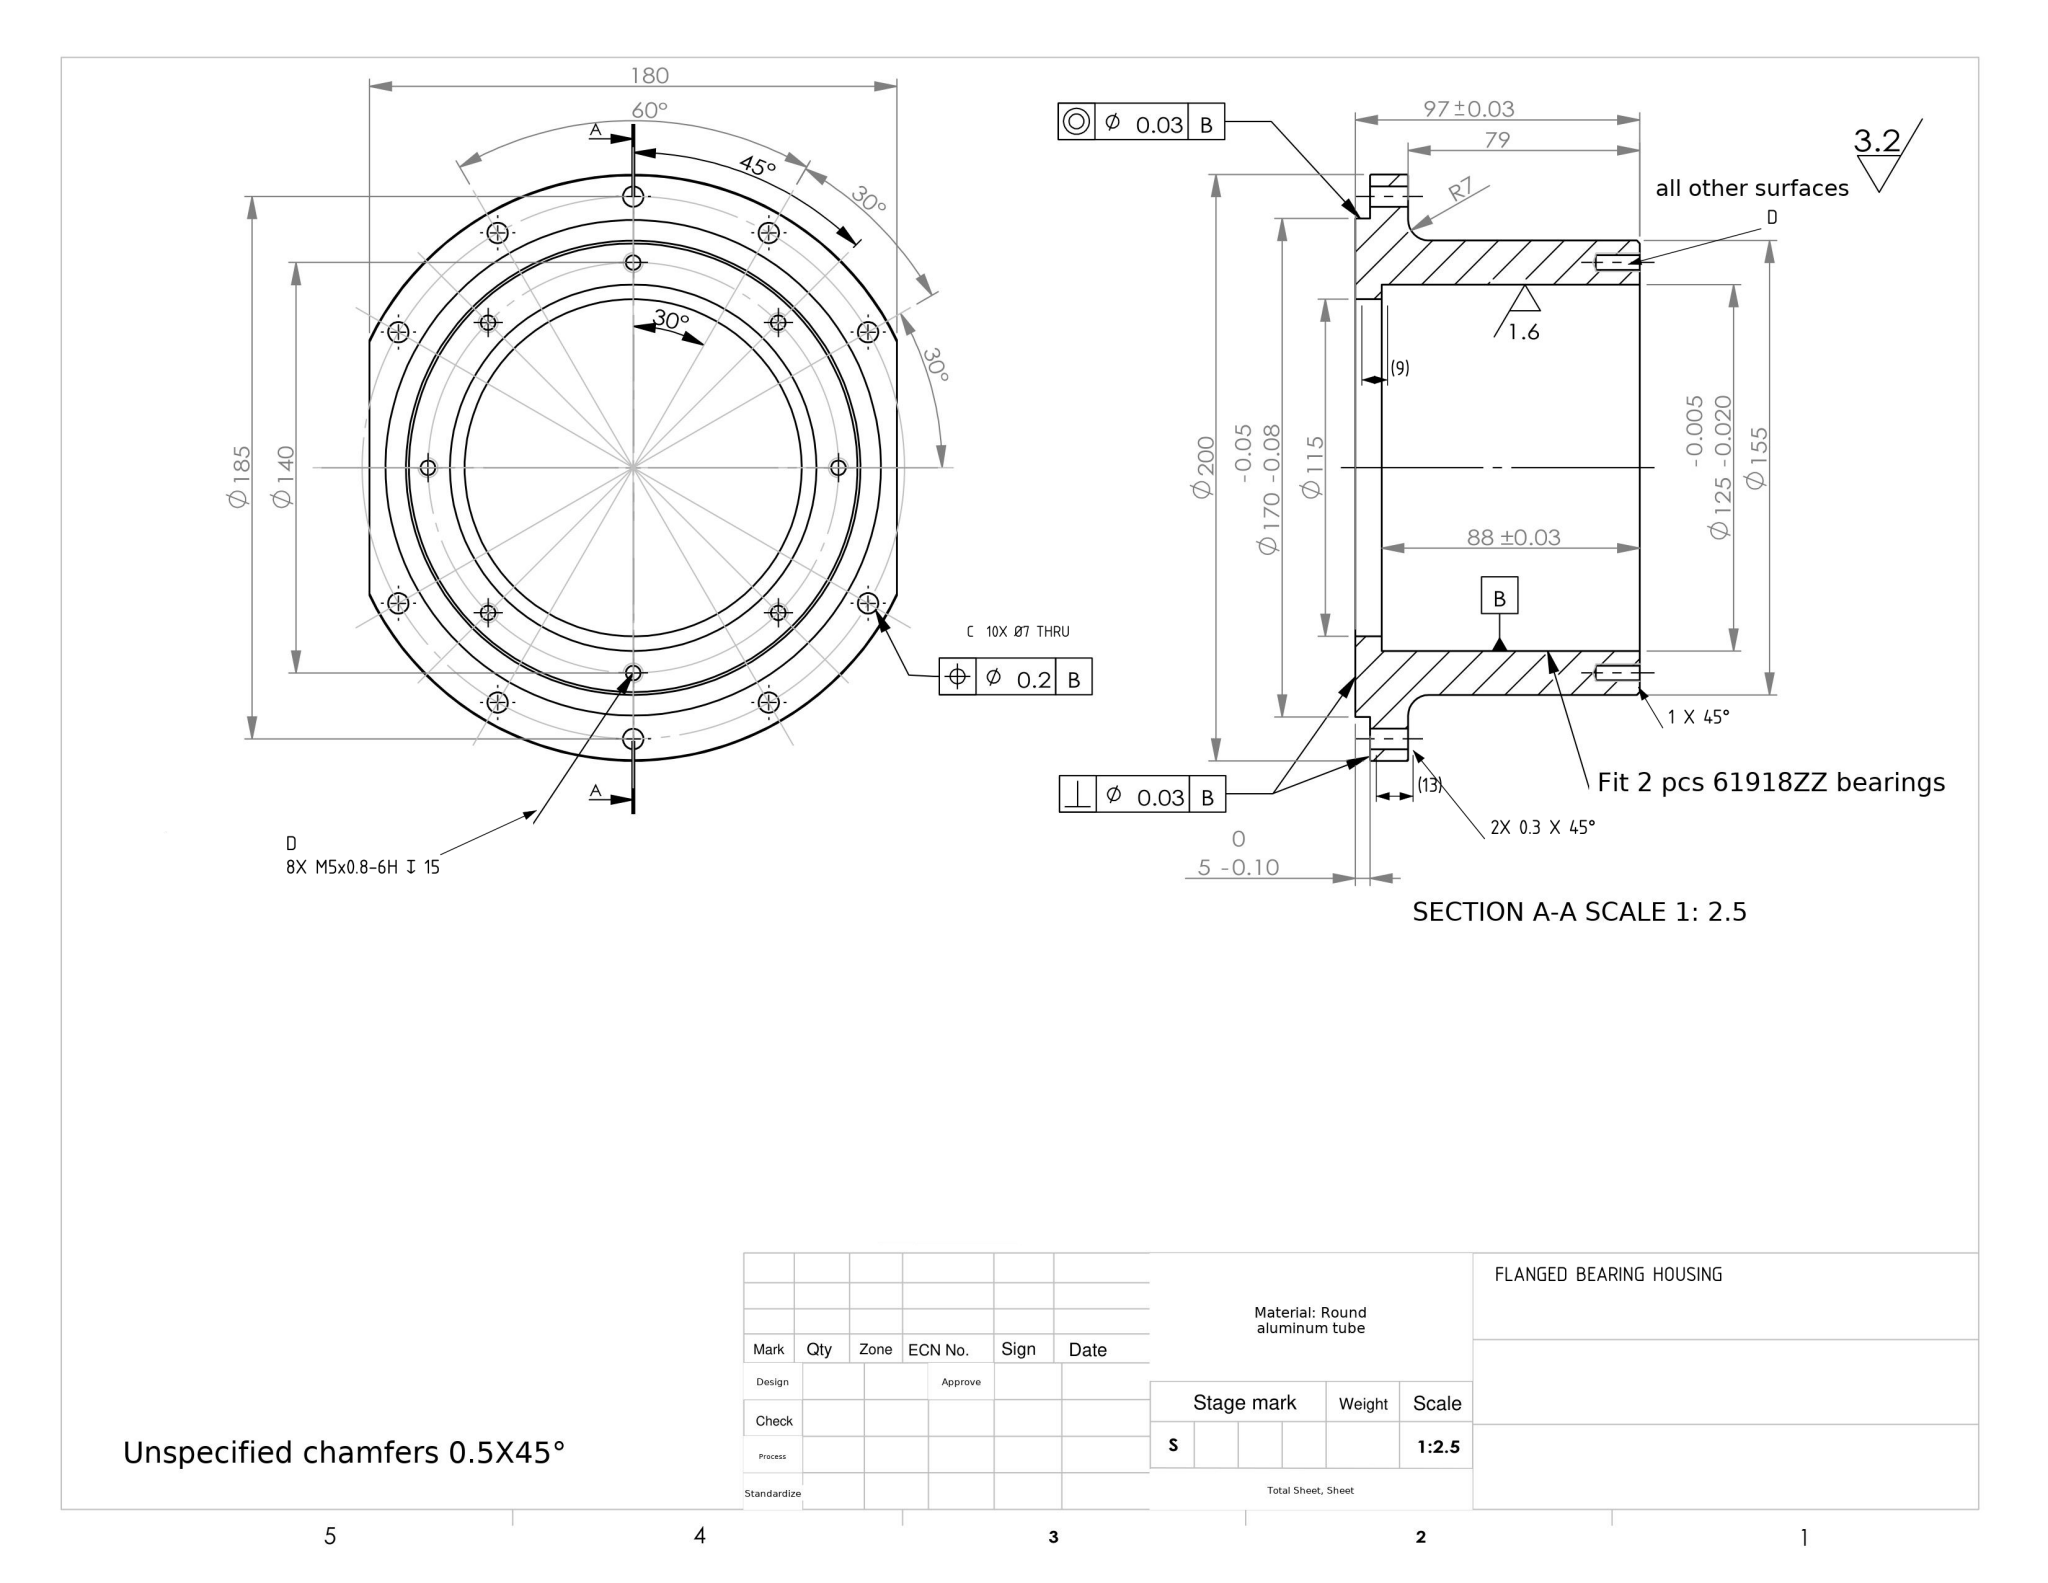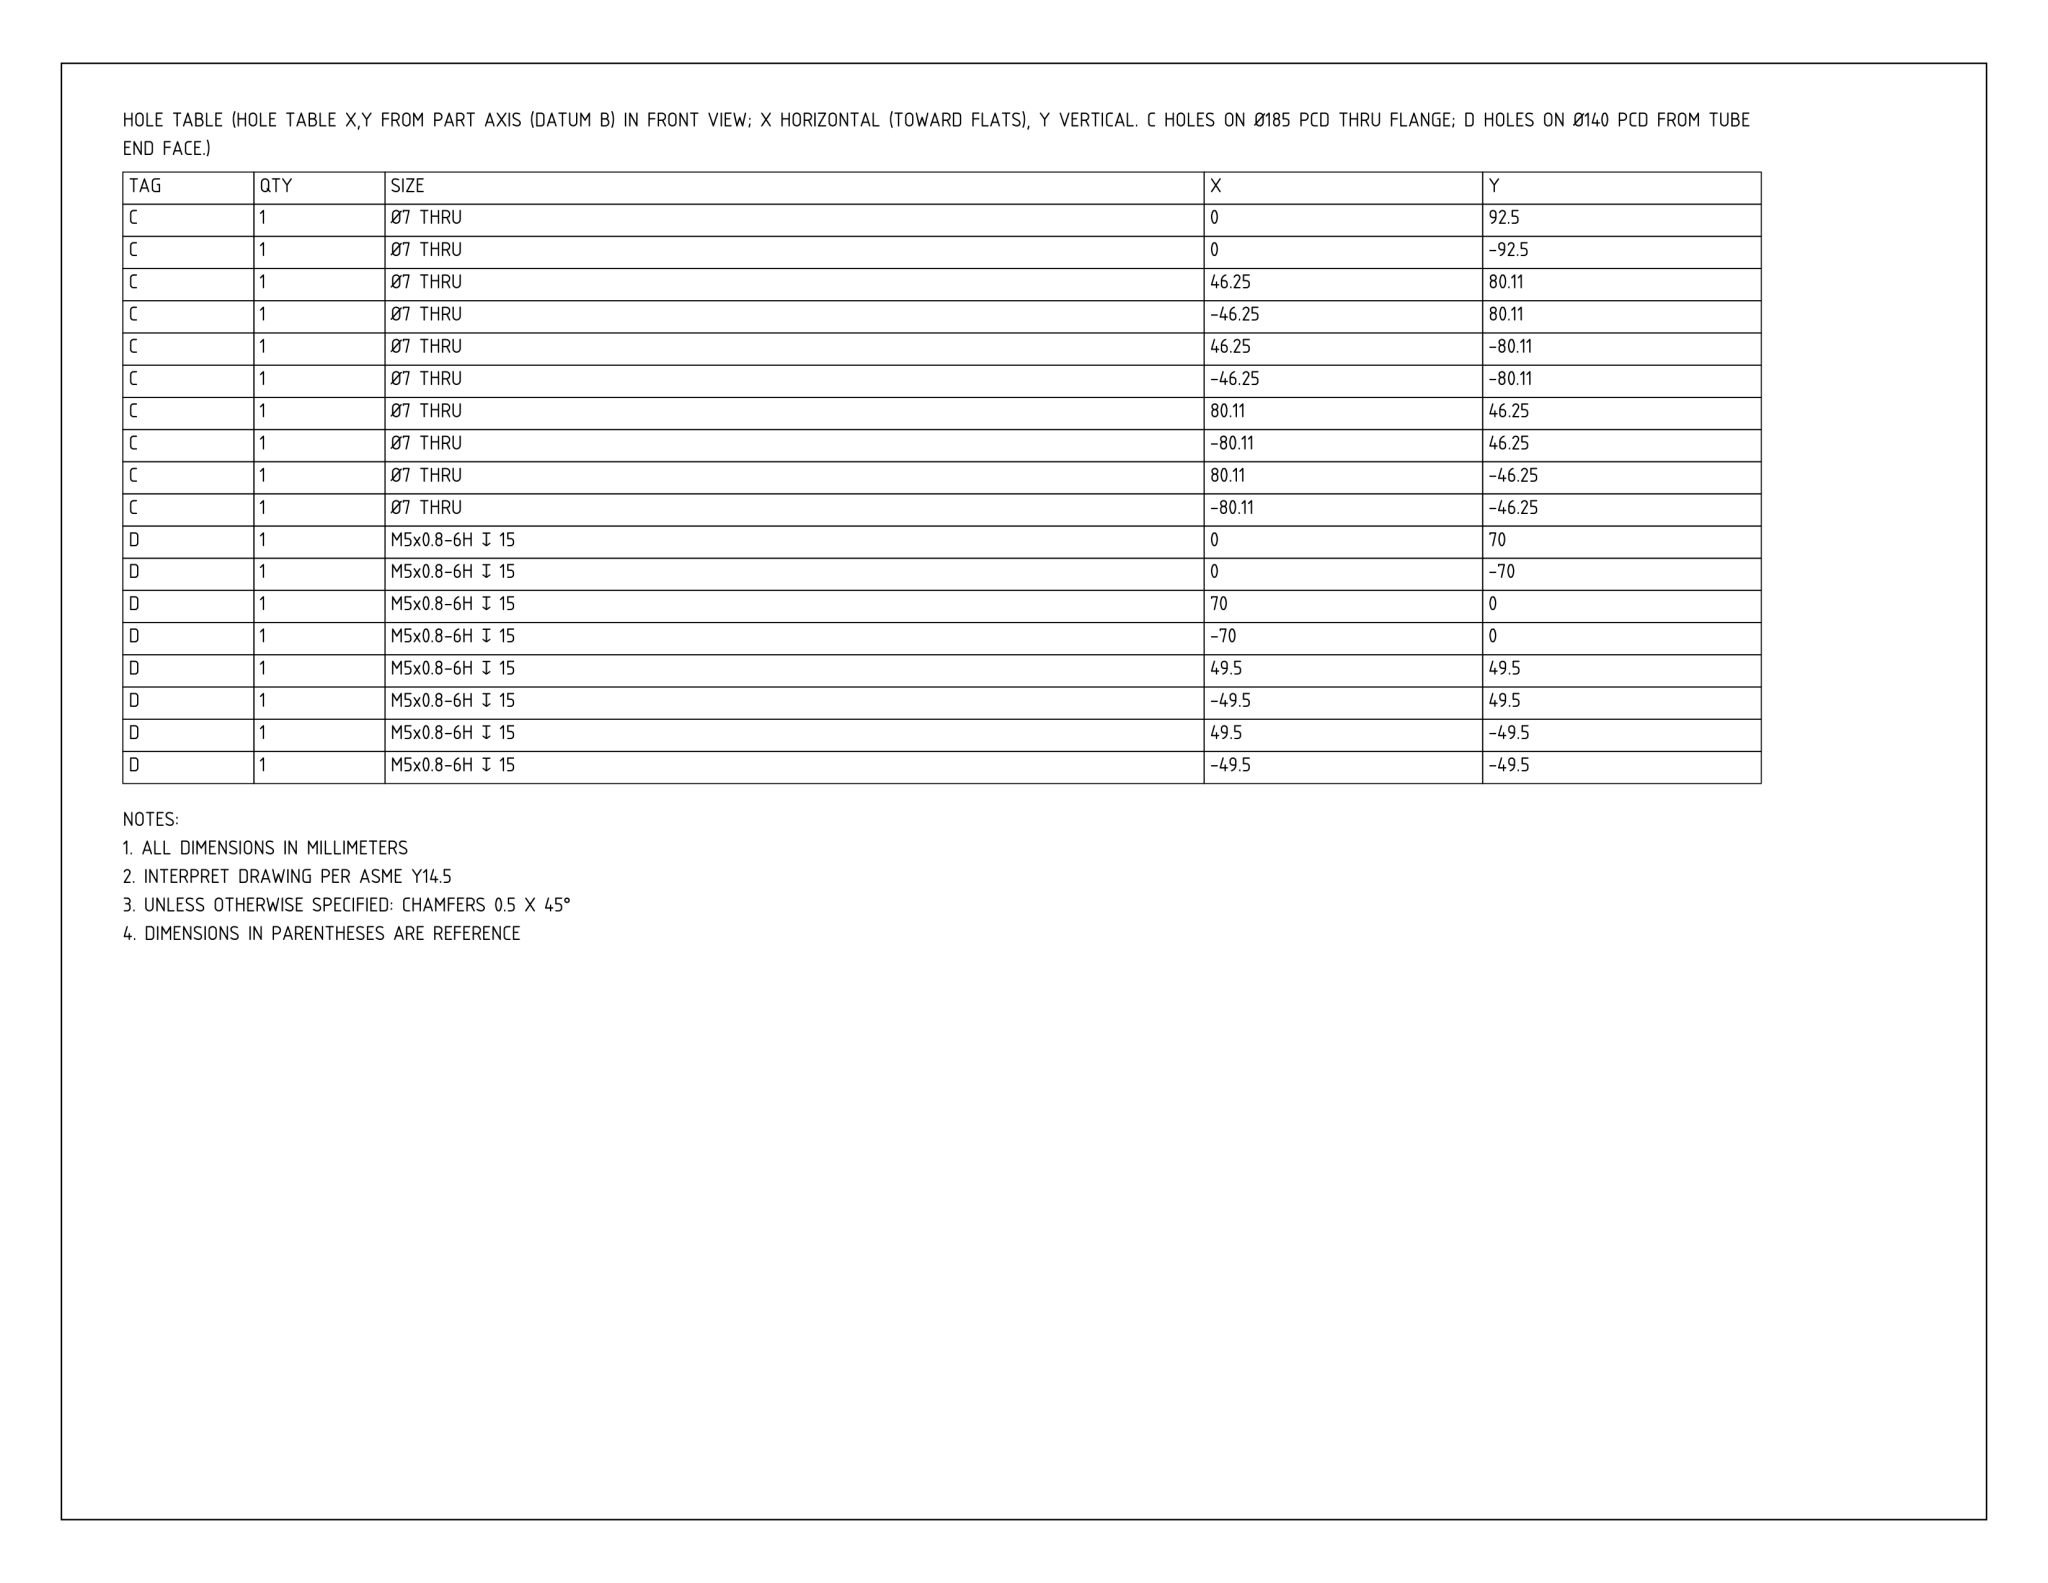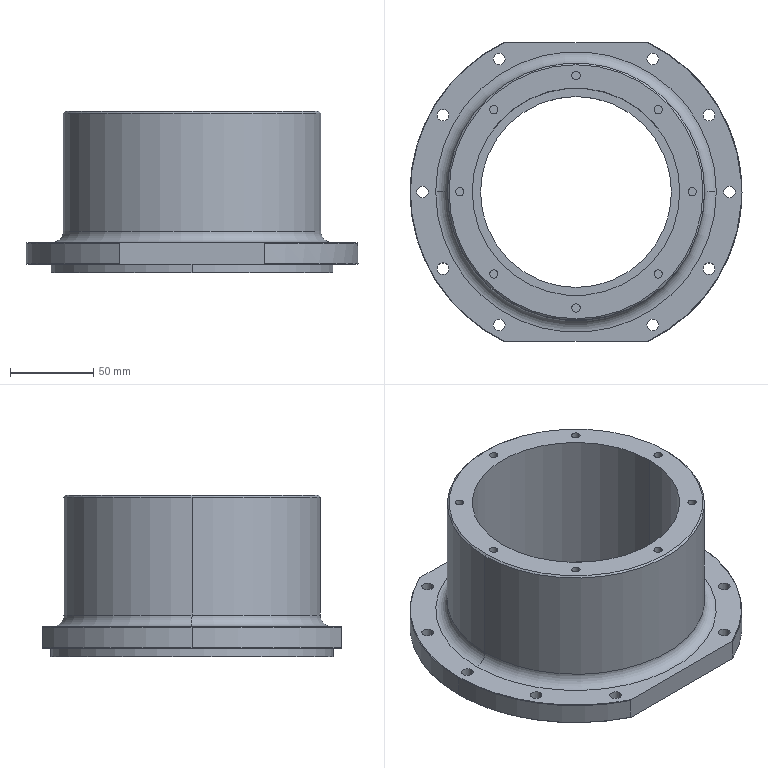Part | NX | mm | 1 solid | 72 faces | box 200 x 180 x 97 mm | volume 821472 mm3 | cylinder 47 | plane 15 | cone 8 | torus 2 | commonest cylinder face diameters 7 x20 5 x16 200 x3 115 x2 170 x2 155 x2 125 x2